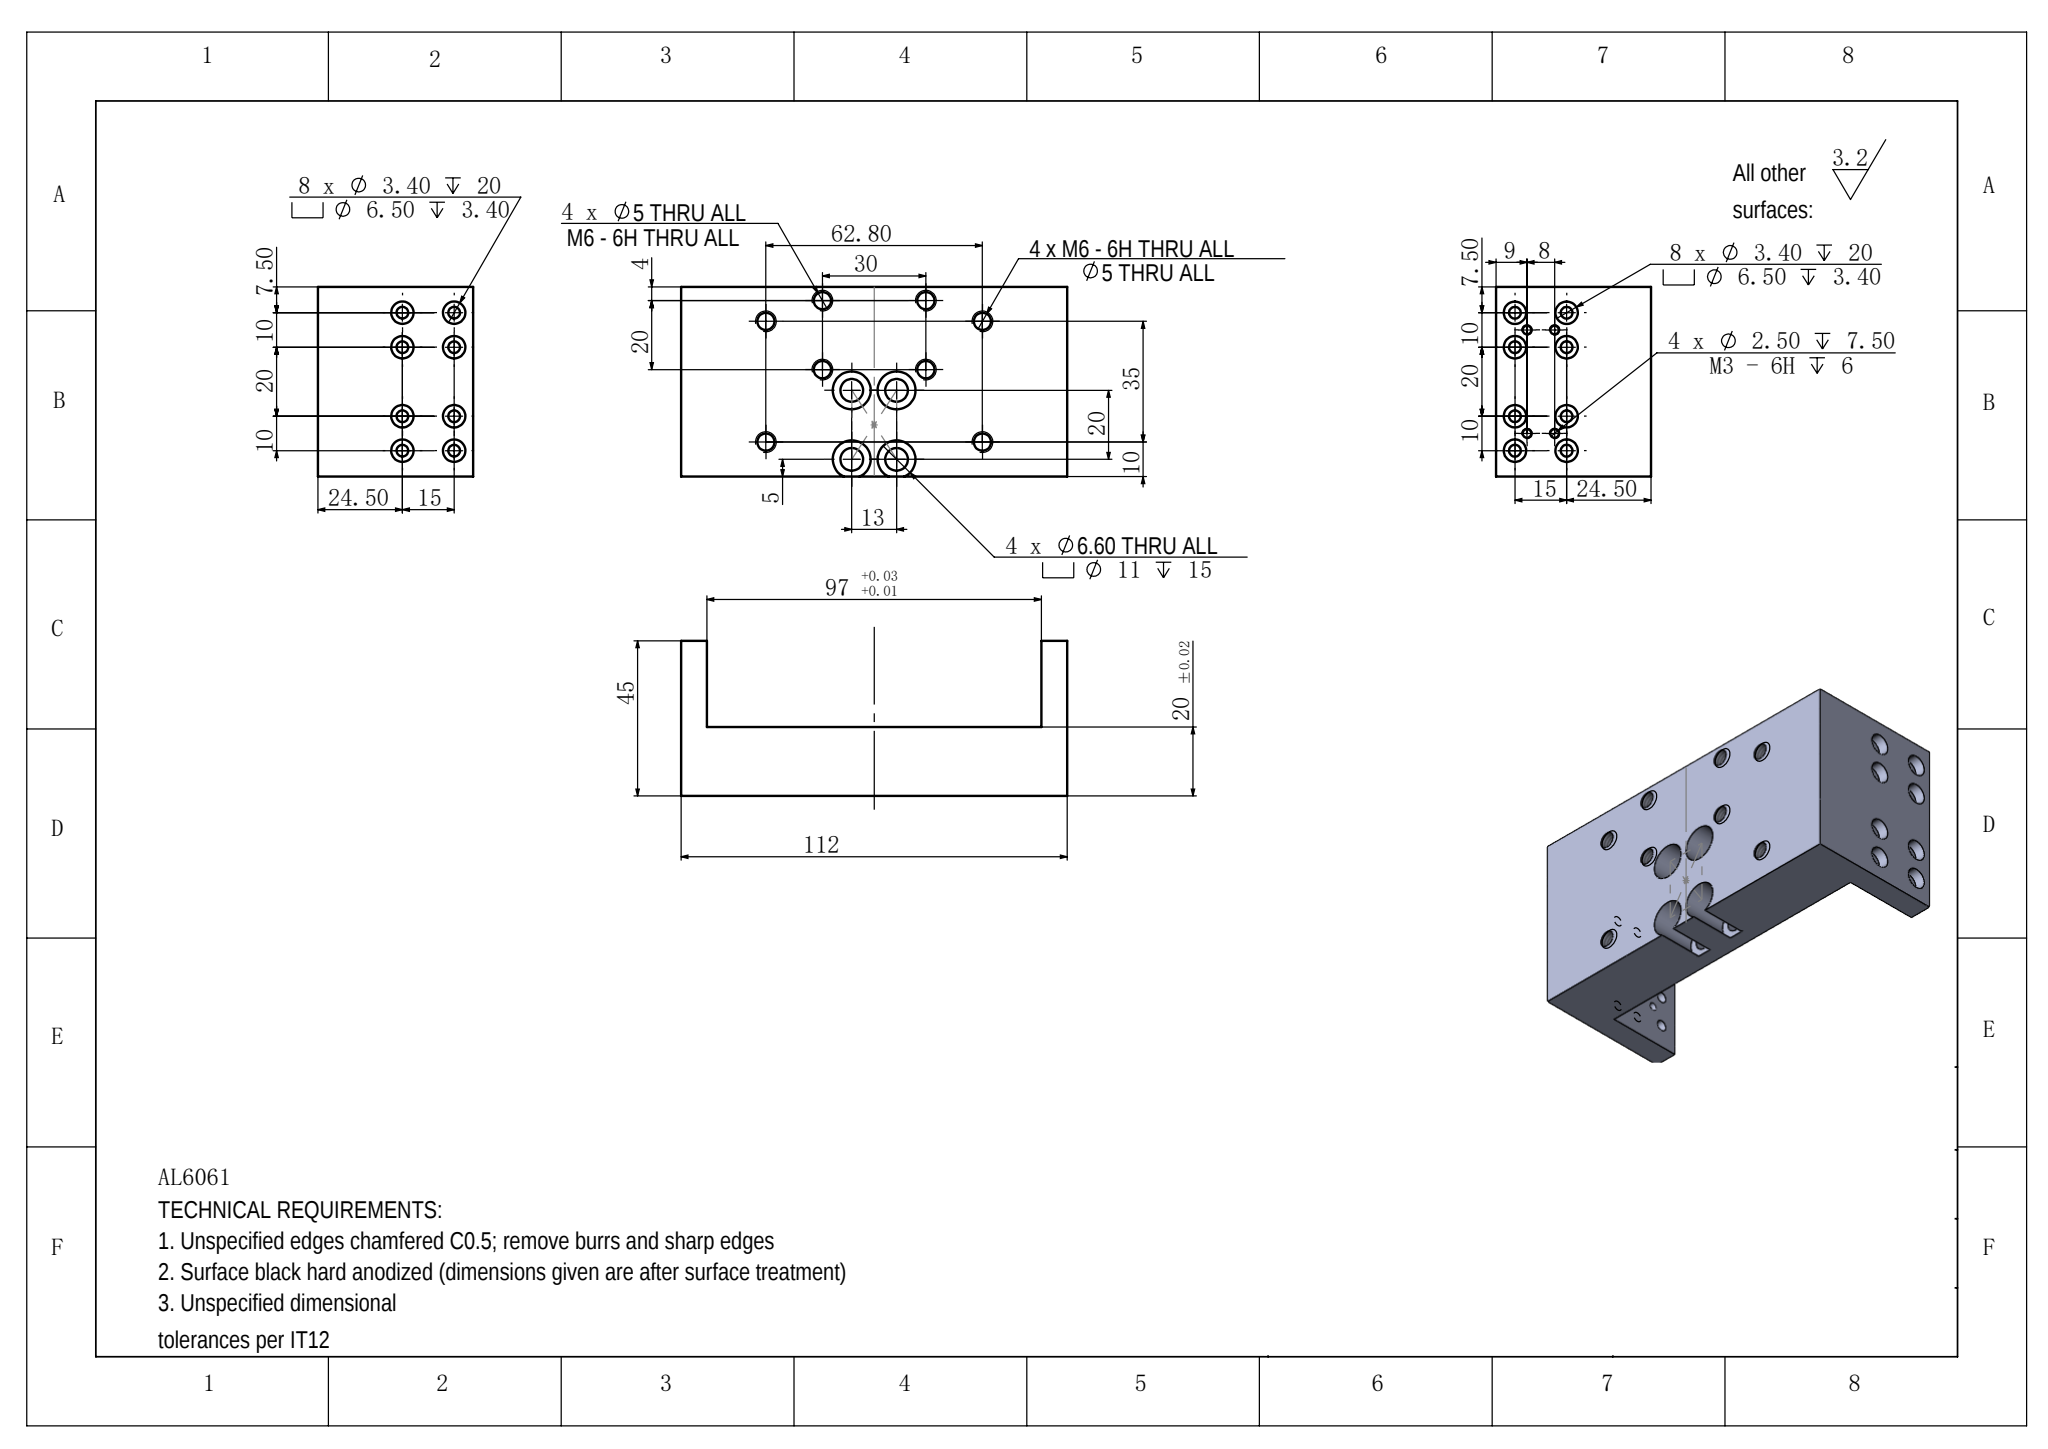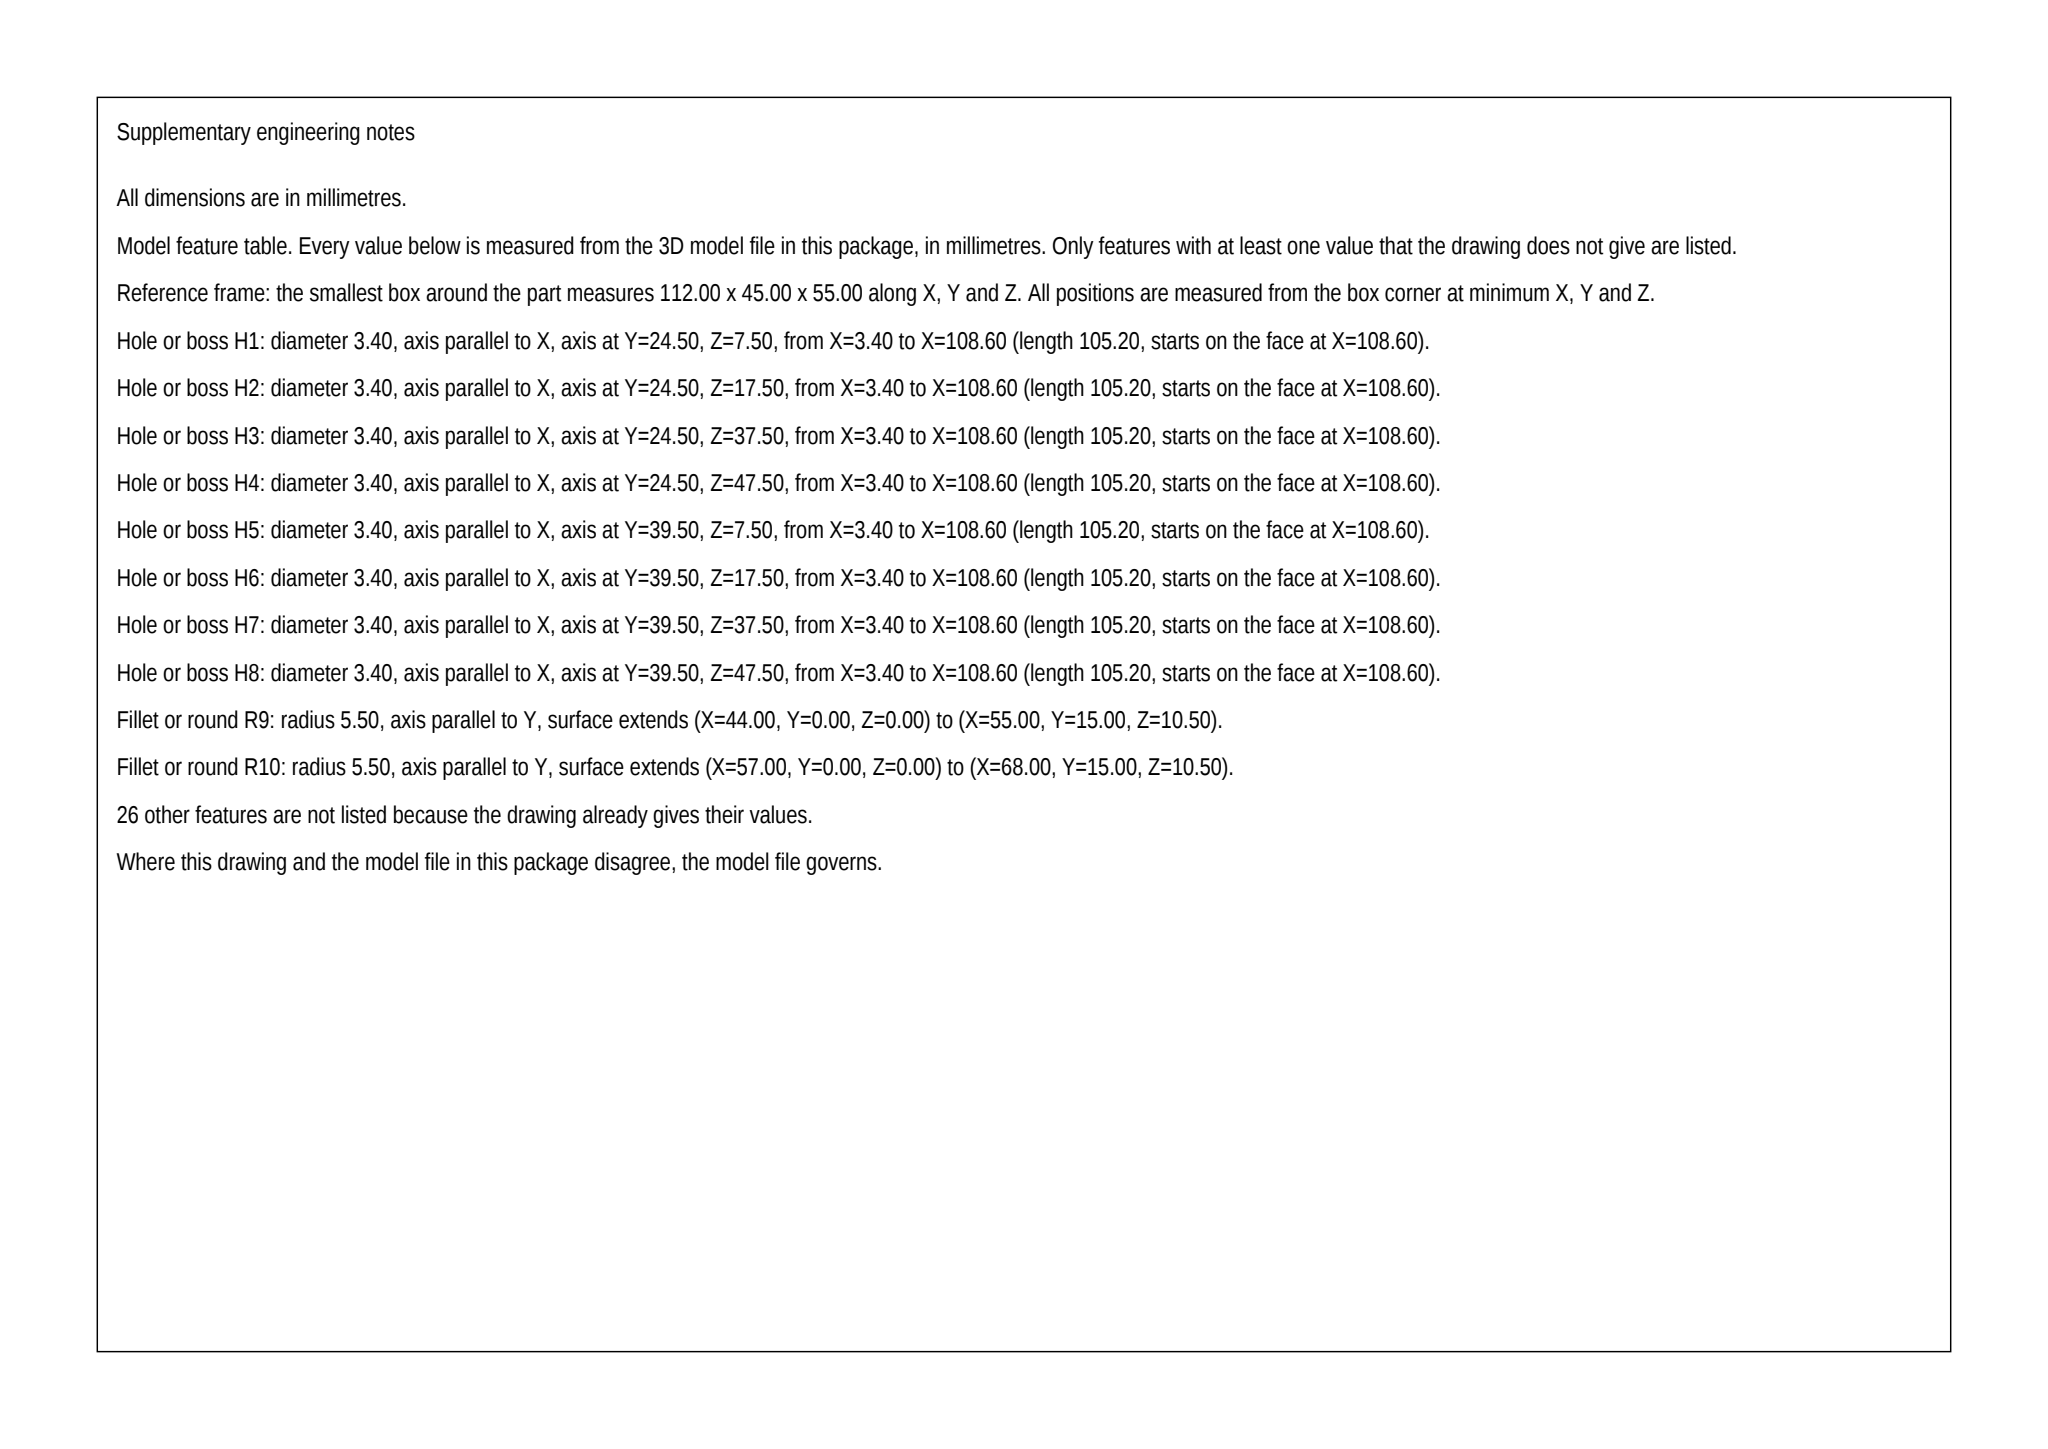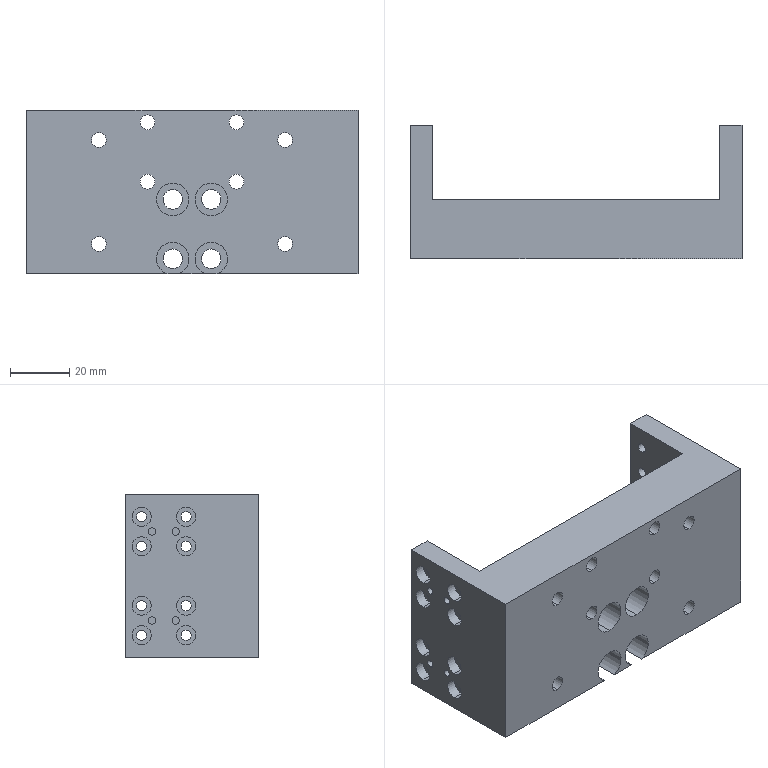Part | SolidWorks | mm | 1 solid | 132 faces | box 112 x 45 x 55 mm | volume 131795 mm3 | cylinder 102 | plane 30 | commonest cylinder face diameters 6.5 x32 3.4 x32 5 x16 2.5 x8 6.6 x8 11 x6
Drawing notes:
8X Ø2.50 DP 7.50, M3-6H DP 6 - 4 holes in each end face (X=0 and X=112), at Y=28 & 36, Z=12.50 & 42.50 from bbox min corner | from the solid: cylinders dia 2.5, axis x, pos (y=28/36, z=12.5/42.5), length 7.5, count 2 each (8 total)
4X Ø6.60 THRU (5 thk web), C'BORE Ø11 DP 15 - holes at X=49.50 & 62.50, Z=5.00 & 25.00 from bbox min corner | from the solid: cylinders dia 6.6 axis y length 5 and dia 11 axis y length 15 at x=49.5/62.5, z=5/25
Ø11 DP 15 counterbore is machined from the underside face Y=0; remaining Ø6.60 breaks through at Y=20 face (15 + 5 = 20 plate thickness) | from the solid: axis_planes y=0, y=15, y=20; dia 11 length 15 and dia 6.6 length 5 share axes at x=49.5/62.5
Overall size 112 (X) x 45 (Y) x 55 (Z) | from the solid: bbox_xyz [112.0, 45.0, 55.0]
All dimensions in millimetres (mm) | from the solid: STEP model facts stated in mm
build123d program:
from build123d import *

# Parameters (mm, degrees)
BOSS_EXTRUDE1_DEPTH                               = 27.5
HOLE_SIZE_ACCORDING_TO_HEXALOBULAR_SO_D           = 6.6
HOLE_SIZE_ACCORDING_TO_HEXALOBULAR_SO_CBORE_D     = 11
HOLE_SIZE_ACCORDING_TO_HEXALOBULAR_SO_CBORE_DEPTH = 15
M6_TAPPED_HOLE1_D                                 = 5
M3_HEX_SOCKET_HEAD_CAP_SCREW_CBORE1_AT_2_COUNT    = 2
M3_HEX_SOCKET_HEAD_CAP_SCREW_CBORE1_AT_2_PITCH    = 15
M3_HEX_SOCKET_HEAD_CAP_SCREW_CBORE1_AT_3_COUNT    = 2
M3_HEX_SOCKET_HEAD_CAP_SCREW_CBORE1_AT_3_PITCH    = 10
M3_HEX_SOCKET_HEAD_CAP_SCREW_CBORE1_AT_4_COUNT    = 2
M3_HEX_SOCKET_HEAD_CAP_SCREW_CBORE1_AT_4_PITCH    = 18.028
M3_HEX_SOCKET_HEAD_CAP_SCREW_CBORE1_AT_5_COUNT    = 2
M3_HEX_SOCKET_HEAD_CAP_SCREW_CBORE1_AT_5_PITCH    = 30
M3_HEX_SOCKET_HEAD_CAP_SCREW_CBORE1_AT_6_COUNT    = 2
M3_HEX_SOCKET_HEAD_CAP_SCREW_CBORE1_AT_6_PITCH    = 33.541
M3_HEX_SOCKET_HEAD_CAP_SCREW_CBORE1_AT_7_COUNT    = 2
M3_HEX_SOCKET_HEAD_CAP_SCREW_CBORE1_AT_7_PITCH    = 40
M3_HEX_SOCKET_HEAD_CAP_SCREW_CBORE1_AT_8_COUNT    = 2
M3_HEX_SOCKET_HEAD_CAP_SCREW_CBORE1_AT_8_PITCH    = 42.72
M3_TAPPED_HOLE1_D                                 = 2.5
M3_TAPPED_HOLE1_DEPTH                             = 7.5
M3_TAPPED_HOLE1_TIP                               = 0.7511
M6_TAPPED_HOLE2_D                                 = 5


with BuildPart() as part:
    # Sketch1 → Boss-Extrude1 (new, symmetric)
    with BuildSketch(Plane.XY):
        Polygon((-56, 45), (-56, 0), (56, 0), (56, 45), (48.5, 45), (48.5, 20), (-48.5, 20), (-48.5, 45), align=None)
    extrude(amount=BOSS_EXTRUDE1_DEPTH, both=True)

    # Hole Size _ according to_ Hexalobular So (through all)
    with Locations(Plane(origin=(0, 0, 0), x_dir=(-1, 0, 0), z_dir=(0, -1, 0))):
        with Locations((6.5, 2.5), (6.5, 22.5), (-6.5, 2.5), (-6.5, 22.5)):
            CounterBoreHole(HOLE_SIZE_ACCORDING_TO_HEXALOBULAR_SO_D / 2, HOLE_SIZE_ACCORDING_TO_HEXALOBULAR_SO_CBORE_D / 2, HOLE_SIZE_ACCORDING_TO_HEXALOBULAR_SO_CBORE_DEPTH)

    # M6 Tapped Hole1 (through all)
    with Locations(Plane(origin=(0, 0, 0), x_dir=(-1, 0, 0), z_dir=(0, -1, 0))):
        with Locations((31.4, -17.5), (31.4, 17.5), (-31.4, -17.5), (-31.4, 17.5)):
            Hole(M6_TAPPED_HOLE1_D / 2)

    # Sketch8 → M3 Hex Socket Head Cap Screw CBORE1 (revolve, cut)
    with BuildSketch(Plane(origin=(-56, 24.5, 20), x_dir=(0, 0, 1), z_dir=(0, 1, 0))):
        Polygon((0, 0), (0, 21.021), (1.7, 20), (1.7, 3.4), (3.25, 3.4), (3.25, 0), align=None)
    m3_hex_socket_head_cap_screw_cbore1 = revolve(axis=Axis((-62.35, 24.5, 20), (1, 0, 0)), mode=Mode.SUBTRACT)

    # M3 Hex Socket Head Cap Screw CBORE1 at 2: M3 Hex Socket Head Cap Screw CBORE1 ×2
    with Locations(*[(0, i * M3_HEX_SOCKET_HEAD_CAP_SCREW_CBORE1_AT_2_PITCH, 0) for i in range(1, M3_HEX_SOCKET_HEAD_CAP_SCREW_CBORE1_AT_2_COUNT)]):
        add(m3_hex_socket_head_cap_screw_cbore1, mode=Mode.SUBTRACT)

    # M3 Hex Socket Head Cap Screw CBORE1 at 3: M3 Hex Socket Head Cap Screw CBORE1 ×2
    with Locations(*[(0, 0, -i * M3_HEX_SOCKET_HEAD_CAP_SCREW_CBORE1_AT_3_PITCH) for i in range(1, M3_HEX_SOCKET_HEAD_CAP_SCREW_CBORE1_AT_3_COUNT)]):
        add(m3_hex_socket_head_cap_screw_cbore1, mode=Mode.SUBTRACT)

    # M3 Hex Socket Head Cap Screw CBORE1 at 4: M3 Hex Socket Head Cap Screw CBORE1 ×2
    with Locations(*[Vector(0, 0.8321, -0.5547) * (i * M3_HEX_SOCKET_HEAD_CAP_SCREW_CBORE1_AT_4_PITCH) for i in range(1, M3_HEX_SOCKET_HEAD_CAP_SCREW_CBORE1_AT_4_COUNT)]):
        add(m3_hex_socket_head_cap_screw_cbore1, mode=Mode.SUBTRACT)

    # M3 Hex Socket Head Cap Screw CBORE1 at 5: M3 Hex Socket Head Cap Screw CBORE1 ×2
    with Locations(*[(0, 0, -i * M3_HEX_SOCKET_HEAD_CAP_SCREW_CBORE1_AT_5_PITCH) for i in range(1, M3_HEX_SOCKET_HEAD_CAP_SCREW_CBORE1_AT_5_COUNT)]):
        add(m3_hex_socket_head_cap_screw_cbore1, mode=Mode.SUBTRACT)

    # M3 Hex Socket Head Cap Screw CBORE1 at 6: M3 Hex Socket Head Cap Screw CBORE1 ×2
    with Locations(*[Vector(0, 0.4472, -0.8944) * (i * M3_HEX_SOCKET_HEAD_CAP_SCREW_CBORE1_AT_6_PITCH) for i in range(1, M3_HEX_SOCKET_HEAD_CAP_SCREW_CBORE1_AT_6_COUNT)]):
        add(m3_hex_socket_head_cap_screw_cbore1, mode=Mode.SUBTRACT)

    # M3 Hex Socket Head Cap Screw CBORE1 at 7: M3 Hex Socket Head Cap Screw CBORE1 ×2
    with Locations(*[(0, 0, -i * M3_HEX_SOCKET_HEAD_CAP_SCREW_CBORE1_AT_7_PITCH) for i in range(1, M3_HEX_SOCKET_HEAD_CAP_SCREW_CBORE1_AT_7_COUNT)]):
        add(m3_hex_socket_head_cap_screw_cbore1, mode=Mode.SUBTRACT)

    # M3 Hex Socket Head Cap Screw CBORE1 at 8: M3 Hex Socket Head Cap Screw CBORE1 ×2
    with Locations(*[Vector(0, 0.3511, -0.9363) * (i * M3_HEX_SOCKET_HEAD_CAP_SCREW_CBORE1_AT_8_PITCH) for i in range(1, M3_HEX_SOCKET_HEAD_CAP_SCREW_CBORE1_AT_8_COUNT)]):
        add(m3_hex_socket_head_cap_screw_cbore1, mode=Mode.SUBTRACT)

    # Mirror1: M3 Hex Socket Head Cap Screw CBORE1 across plane
    add(m3_hex_socket_head_cap_screw_cbore1.mirror(Plane(origin=(0, 0, 0), x_dir=(0, 0, 1), z_dir=(1, 0, 0))), mode=Mode.SUBTRACT)

    # Mirror1 copy 1 sketch → Mirror1 copy 1 (revolve, cut)
    with BuildSketch(Plane(origin=(56, 39.5, 20), x_dir=(0, 0, 1), z_dir=(0, 1, 0))):
        Polygon((0, 0), (0, -21.021), (1.7, -20), (1.7, -3.4), (3.25, -3.4), (3.25, 0), align=None)
    revolve(axis=Axis((62.35, 39.5, 20), (1, 0, 0)), mode=Mode.SUBTRACT)

    # Mirror1 copy 2 sketch → Mirror1 copy 2 (revolve, cut)
    with BuildSketch(Plane(origin=(56, 24.5, 10), x_dir=(0, 0, 1), z_dir=(0, 1, 0))):
        Polygon((0, 0), (0, -21.021), (1.7, -20), (1.7, -3.4), (3.25, -3.4), (3.25, 0), align=None)
    revolve(axis=Axis((62.35, 24.5, 10), (1, 0, 0)), mode=Mode.SUBTRACT)

    # Mirror1 copy 3 sketch → Mirror1 copy 3 (revolve, cut)
    with BuildSketch(Plane(origin=(56, 39.5, 10), x_dir=(0, 0, 1), z_dir=(0, 1, 0))):
        Polygon((0, 0), (0, -21.021), (1.7, -20), (1.7, -3.4), (3.25, -3.4), (3.25, 0), align=None)
    revolve(axis=Axis((62.35, 39.5, 10), (1, 0, 0)), mode=Mode.SUBTRACT)

    # Mirror1 copy 4 sketch → Mirror1 copy 4 (revolve, cut)
    with BuildSketch(Plane(origin=(56, 24.5, -10), x_dir=(0, 0, 1), z_dir=(0, 1, 0))):
        Polygon((0, 0), (0, -21.021), (1.7, -20), (1.7, -3.4), (3.25, -3.4), (3.25, 0), align=None)
    revolve(axis=Axis((62.35, 24.5, -10), (1, 0, 0)), mode=Mode.SUBTRACT)

    # Mirror1 copy 5 sketch → Mirror1 copy 5 (revolve, cut)
    with BuildSketch(Plane(origin=(56, 39.5, -10), x_dir=(0, 0, 1), z_dir=(0, 1, 0))):
        Polygon((0, 0), (0, -21.021), (1.7, -20), (1.7, -3.4), (3.25, -3.4), (3.25, 0), align=None)
    revolve(axis=Axis((62.35, 39.5, -10), (1, 0, 0)), mode=Mode.SUBTRACT)

    # Mirror1 copy 6 sketch → Mirror1 copy 6 (revolve, cut)
    with BuildSketch(Plane(origin=(56, 24.5, -20), x_dir=(0, 0, 1), z_dir=(0, 1, 0))):
        Polygon((0, 0), (0, -21.021), (1.7, -20), (1.7, -3.4), (3.25, -3.4), (3.25, 0), align=None)
    revolve(axis=Axis((62.35, 24.5, -20), (1, 0, 0)), mode=Mode.SUBTRACT)

    # Mirror1 copy 7 sketch → Mirror1 copy 7 (revolve, cut)
    with BuildSketch(Plane(origin=(56, 39.5, -20), x_dir=(0, 0, 1), z_dir=(0, 1, 0))):
        Polygon((0, 0), (0, -21.021), (1.7, -20), (1.7, -3.4), (3.25, -3.4), (3.25, 0), align=None)
    revolve(axis=Axis((62.35, 39.5, -20), (1, 0, 0)), mode=Mode.SUBTRACT)

    # M3 Tapped Hole1
    with Locations(Plane.ZY.offset(56)):
        with Locations((15, 36), (15, 28), (-15, 28), (-15, 36)):
            Hole(M3_TAPPED_HOLE1_D / 2, depth=M3_TAPPED_HOLE1_DEPTH)
            with Locations((0, 0, -(M3_TAPPED_HOLE1_DEPTH + M3_TAPPED_HOLE1_TIP / 2))):  # 118° drill point
                Cone(0, M3_TAPPED_HOLE1_D / 2, M3_TAPPED_HOLE1_TIP, mode=Mode.SUBTRACT)

    # M6 Tapped Hole2 (through all)
    with Locations(Plane(origin=(0, 0, 0), x_dir=(-1, 0, 0), z_dir=(0, -1, 0))):
        with Locations((15, -23.5), (15, -3.5), (-15, -23.5), (-15, -3.5)):
            Hole(M6_TAPPED_HOLE2_D / 2)


solid = part.part